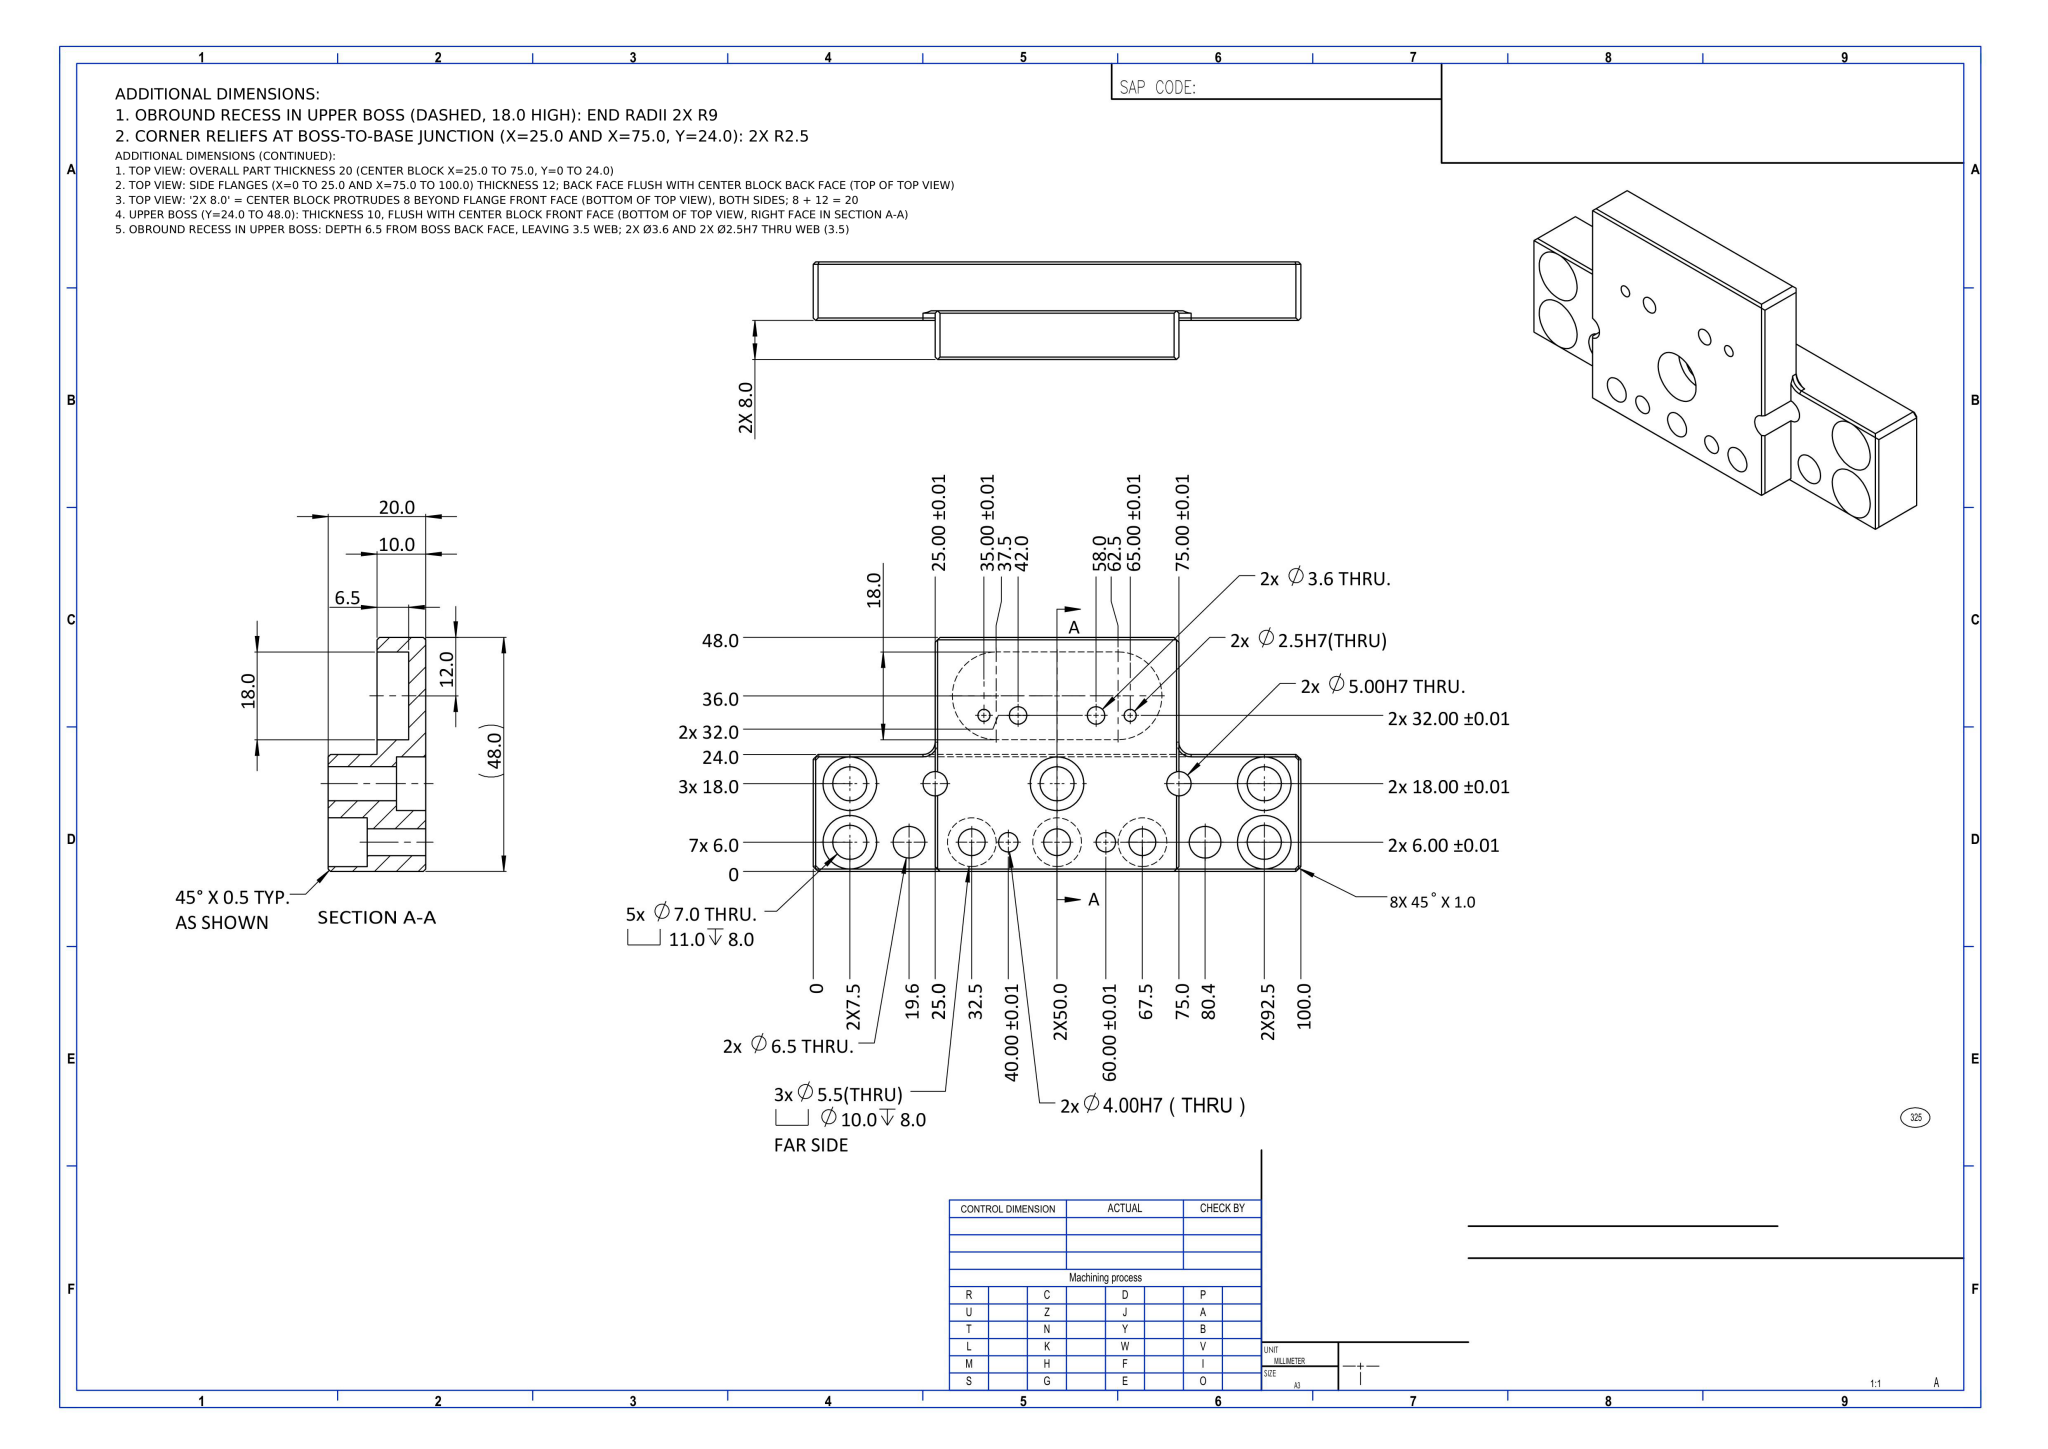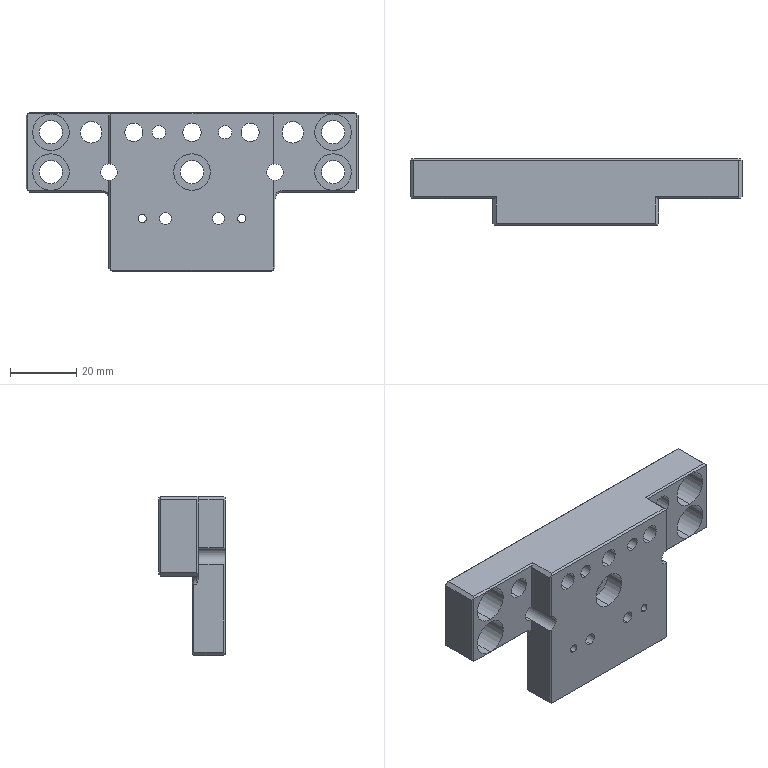Part | NX | mm | 1 solid | 116 faces | box 100 x 20 x 48 mm | volume 36162 mm3 | cylinder 56 | plane 56 | cone 4 | commonest cylinder face diameters 11 x10 7 x10 5 x6 10 x6 5.5 x6 6.5 x4 4 x4 3.6 x4